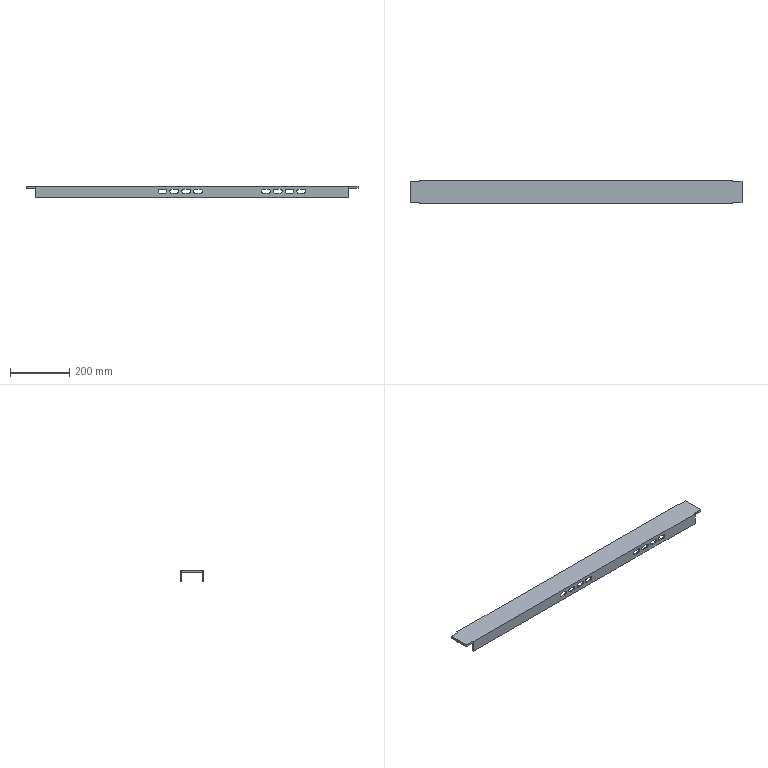Component | SolidWorks | BaseAssembly-1_ChannelSteelAssembly-1_8#ChannelSteel3-1 | 1 solid | 98 faces | box 1124 x 80 x 40 mm | volume 962436 mm3 | plane 50 | cylinder 48 | commonest cylinder face diameters 14 x48
build123d program:
from build123d import *

# Parameters (mm, degrees)
EXTRUDE1_DEPTH         = 1124
SKETCH2_W              = 32
SKETCH2_H              = 32
CUT_EXTRUDE1_DEPTH     = 1128.553
SKETCH3_W              = 32
SKETCH3_H              = 4
CUT_EXTRUDE2_DEPTH     = 1200
CUT_EXTRUDE3_DEPTH     = 1128.553
LPATTERN1_COUNT        = 4
LPATTERN1_PITCH        = 40
LPATTERN2_COUNT        = 2
LPATTERN2_PITCH        = 350
LPATTERN2_COPY_1_DEPTH = 1128.553
LPATTERN2_COPY_2_DEPTH = 1128.553
LPATTERN2_COPY_3_DEPTH = 1128.553


with BuildPart() as part:
    # Sketch1 → Extrude1 (new body)
    with BuildSketch(Plane.XY):
        Polygon((0, 0), (-40, 0), (-40, 80), (0, 80), (0, 76), (-32, 76), (-32, 4), (0, 4), align=None)
    extrude(amount=EXTRUDE1_DEPTH)

    # Sketch2 → Cut-Extrude1 (cut, through all)
    with BuildSketch(Plane(origin=(0, 80, 0), x_dir=(1, 0, 0), z_dir=(0, 1, 0))):
        with Locations((-16, -16)):
            Rectangle(SKETCH2_W, SKETCH2_H)
        with Locations((-16, -1108)):
            Rectangle(SKETCH2_W, SKETCH2_H)
    extrude(amount=-CUT_EXTRUDE1_DEPTH, mode=Mode.SUBTRACT)

    # Sketch3 → Cut-Extrude2 (cut)
    with BuildSketch(Plane(origin=(-32, 0, 0), x_dir=(0, 0, -1), z_dir=(1, 0, 0))):
        with Locations((-1108, 78)):
            Rectangle(SKETCH3_W, SKETCH3_H)
        with Locations((-1108, 2)):
            Rectangle(SKETCH3_W, SKETCH3_H)
        with Locations((-16, 78)):
            Rectangle(SKETCH3_W, SKETCH3_H)
        with Locations((-16, 2)):
            Rectangle(SKETCH3_W, SKETCH3_H)
    extrude(amount=-CUT_EXTRUDE2_DEPTH, mode=Mode.SUBTRACT)

    # Sketch4 → Cut-Extrude3 (cut, through all)
    with BuildSketch(Plane(origin=(0, 80, 0), x_dir=(1, 0, 0), z_dir=(0, 1, 0))):
        with BuildLine():
            Line((-29.5, -924), (-29.5, -940))
            ThreePointArc((-29.5, -940), (-22.5, -947), (-15.5, -940))
            Line((-15.5, -940), (-15.5, -924))
            ThreePointArc((-15.5, -924), (-22.5, -917), (-29.5, -924))
        make_face()
    cut_extrude3 = extrude(amount=-CUT_EXTRUDE3_DEPTH, mode=Mode.SUBTRACT)

    # LPattern1: Cut-Extrude3 ×4
    with Locations(*[(0, 0, -i * LPATTERN1_PITCH) for i in range(1, LPATTERN1_COUNT)]):
        add(cut_extrude3, mode=Mode.SUBTRACT)

    # LPattern2: Cut-Extrude3 ×2
    with Locations(*[(0, 0, -i * LPATTERN2_PITCH) for i in range(1, LPATTERN2_COUNT)]):
        add(cut_extrude3, mode=Mode.SUBTRACT)

    # LPattern2 copy 1 sketch → LPattern2 copy 1 (cut, through all)
    with BuildSketch(Plane(origin=(0, 80, -390), x_dir=(1, 0, 0), z_dir=(0, 1, 0))):
        with BuildLine():
            Line((-29.5, -924), (-29.5, -940))
            ThreePointArc((-29.5, -940), (-22.5, -947), (-15.5, -940))
            Line((-15.5, -940), (-15.5, -924))
            ThreePointArc((-15.5, -924), (-22.5, -917), (-29.5, -924))
        make_face()
    extrude(amount=-LPATTERN2_COPY_1_DEPTH, mode=Mode.SUBTRACT)

    # LPattern2 copy 2 sketch → LPattern2 copy 2 (cut, through all)
    with BuildSketch(Plane(origin=(0, 80, -430), x_dir=(1, 0, 0), z_dir=(0, 1, 0))):
        with BuildLine():
            Line((-29.5, -924), (-29.5, -940))
            ThreePointArc((-29.5, -940), (-22.5, -947), (-15.5, -940))
            Line((-15.5, -940), (-15.5, -924))
            ThreePointArc((-15.5, -924), (-22.5, -917), (-29.5, -924))
        make_face()
    extrude(amount=-LPATTERN2_COPY_2_DEPTH, mode=Mode.SUBTRACT)

    # LPattern2 copy 3 sketch → LPattern2 copy 3 (cut, through all)
    with BuildSketch(Plane(origin=(0, 80, -470), x_dir=(1, 0, 0), z_dir=(0, 1, 0))):
        with BuildLine():
            Line((-29.5, -924), (-29.5, -940))
            ThreePointArc((-29.5, -940), (-22.5, -947), (-15.5, -940))
            Line((-15.5, -940), (-15.5, -924))
            ThreePointArc((-15.5, -924), (-22.5, -917), (-29.5, -924))
        make_face()
    extrude(amount=-LPATTERN2_COPY_3_DEPTH, mode=Mode.SUBTRACT)


solid = part.part

# Placed as in the assembly
solid = solid.moved(Location((-409.218, -82.9, -367.5), (0, 90, 0)))